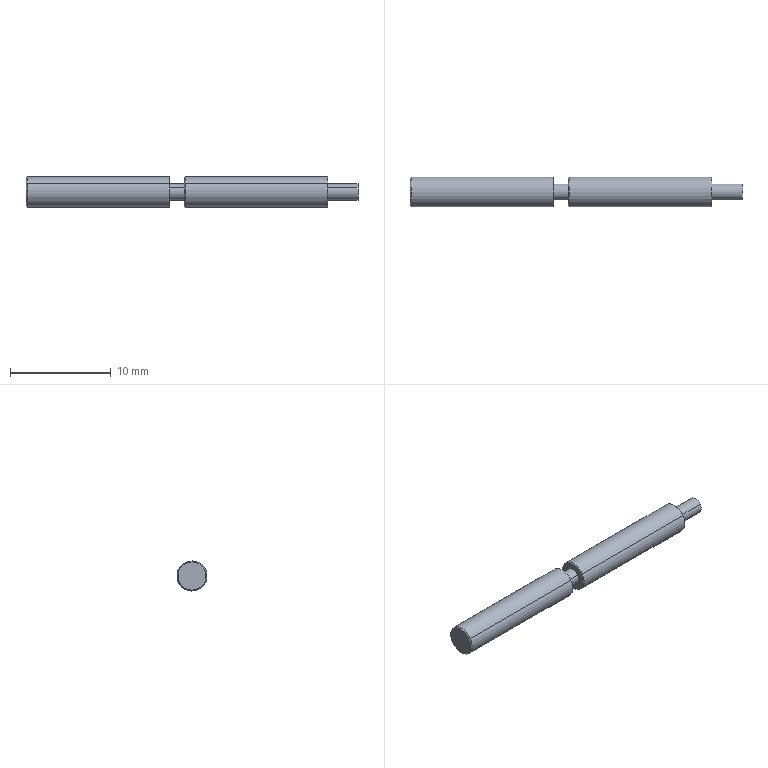Component | SolidWorks | SliderScrew2-1 | 1 solid | 17 faces | box 33 x 3 x 3 mm | volume 210 mm3 | cylinder 8 | plane 5 | cone 4 | commonest cylinder face diameters 1.6 x4 3 x4
build123d program:
from build123d import *

# Parameters (mm, degrees)
SKETCH1_R           = 1.5
BOSS_EXTRUDE1_DEPTH = 15
CHAMFER1_SIZE       = 0.1
SKETCH2_R           = 1.5
SKETCH2_R_2         = 0.8
CUT_EXTRUDE1_DEPTH  = 0.75
CHAMFER2_SIZE       = 0.1
SKETCH3_R           = 0.8
BOSS_EXTRUDE2_DEPTH = 3


with BuildPart() as part:
    # Sketch1 → Boss-Extrude1 (new, symmetric)
    with BuildSketch(Plane.XY):
        Circle(SKETCH1_R)
    extrude(amount=BOSS_EXTRUDE1_DEPTH, both=True)

    # Chamfer1
    chamfer1_edges = [part.edges().sort_by_distance(p)[0] for p in [
        (-1.5, 0, -15),
    ]]
    chamfer(chamfer1_edges, length=CHAMFER1_SIZE)

    # Sketch2 → Cut-Extrude1 (cut, symmetric)
    with BuildSketch(Plane.XY):
        Circle(SKETCH2_R)
        Circle(SKETCH2_R_2, mode=Mode.SUBTRACT)
    extrude(amount=CUT_EXTRUDE1_DEPTH, both=True, mode=Mode.SUBTRACT)

    # Chamfer2
    chamfer2_edges = [part.edges().sort_by_distance(p)[0] for p in [
        (-1.5, 0, 0.75),
    ]]
    chamfer(chamfer2_edges, length=CHAMFER2_SIZE)

    # Sketch3 → Boss-Extrude2 (add)
    with BuildSketch(Plane.XY.offset(15)):
        Circle(SKETCH3_R)
    extrude(amount=BOSS_EXTRUDE2_DEPTH)


solid = part.part

# Placed as in the assembly
solid = solid.moved(Location((-5.981, 33.561, 233.566), (0, 90, 0)))
STEP:
#1=COLOUR_RGB('',0.7922,0.8196,0.9333);
#2=FILL_AREA_STYLE_COLOUR('',#1);
#3=FILL_AREA_STYLE('',(#2));
#4=SURFACE_STYLE_FILL_AREA(#3);
#5=SURFACE_SIDE_STYLE('',(#4));
#6=SURFACE_STYLE_USAGE(.BOTH.,#5);
#7=PRESENTATION_STYLE_ASSIGNMENT((#6));
#8=CARTESIAN_POINT('',(0.4732,1.295,9.213));
#9=VERTEX_POINT('',#8);
#10=CARTESIAN_POINT('',(0.4732,1.347,9.178));
#11=VERTEX_POINT('',#10);
#12=CARTESIAN_POINT('',(0.4732,1.321,9.196));
#13=DIRECTION('',(1.,0.,-0.));
#14=DIRECTION('',(0.,-0.8262,0.5634));
#15=AXIS2_PLACEMENT_3D('',#12,#13,#14);
#16=CIRCLE('',#15,0.0315);
#17=EDGE_CURVE('',#9,#11,#16,.T.);
#18=ORIENTED_EDGE('',*,*,#17,.F.);
#19=CARTESIAN_POINT('',(0.3551,1.295,9.213));
#20=VERTEX_POINT('',#19);
#21=CARTESIAN_POINT('',(0.4732,1.295,9.213));
#22=DIRECTION('',(-1.,-0.,0.));
#23=VECTOR('',#22,39.37);
#24=LINE('',#21,#23);
#25=EDGE_CURVE('',#9,#20,#24,.T.);
#26=ORIENTED_EDGE('',*,*,#25,.T.);
#27=CARTESIAN_POINT('',(0.3551,1.347,9.178));
#28=VERTEX_POINT('',#27);
#29=CARTESIAN_POINT('',(0.3551,1.321,9.196));
#30=DIRECTION('',(1.,0.,-0.));
#31=DIRECTION('',(0.,-0.8262,0.5634));
#32=AXIS2_PLACEMENT_3D('',#29,#30,#31);
#33=CIRCLE('',#32,0.0315);
#34=EDGE_CURVE('',#20,#28,#33,.T.);
#35=ORIENTED_EDGE('',*,*,#34,.T.);
#36=CARTESIAN_POINT('',(0.4732,1.347,9.178));
#37=DIRECTION('',(-1.,-0.,0.));
#38=VECTOR('',#37,39.37);
#39=LINE('',#36,#38);
#40=EDGE_CURVE('',#11,#28,#39,.T.);
#41=ORIENTED_EDGE('',*,*,#40,.F.);
#42=EDGE_LOOP('',(#18,#26,#35,#41));
#43=FACE_OUTER_BOUND('',#42,.T.);
#44=CARTESIAN_POINT('',(0.4732,1.321,9.196));
#45=DIRECTION('',(-1.,-0.,0.));
#46=DIRECTION('',(0.,0.8262,-0.5634));
#47=AXIS2_PLACEMENT_3D('',#44,#45,#46);
#48=CYLINDRICAL_SURFACE('',#47,0.0315);
#49=ADVANCED_FACE('',(#43),#48,.T.);
#50=CARTESIAN_POINT('',(-0.2059,1.367,9.164));
#51=VERTEX_POINT('',#50);
#52=CARTESIAN_POINT('',(-0.2059,1.276,9.227));
#53=VERTEX_POINT('',#52);
#54=CARTESIAN_POINT('',(-0.2059,1.321,9.196));
#55=DIRECTION('',(-1.,-0.,0.));
#56=DIRECTION('',(0.,-0.8262,0.5634));
#57=AXIS2_PLACEMENT_3D('',#54,#55,#56);
#58=CIRCLE('',#57,0.05512);
#59=EDGE_CURVE('',#51,#53,#58,.T.);
#60=ORIENTED_EDGE('',*,*,#59,.F.);
#61=CARTESIAN_POINT('',(-0.202,1.37,9.162));
#62=VERTEX_POINT('',#61);
#63=CARTESIAN_POINT('',(-0.202,1.37,9.162));
#64=DIRECTION('',(0.7071,0.5842,-0.3984));
#65=VECTOR('',#64,39.37);
#66=LINE('',#63,#65);
#67=EDGE_CURVE('',#51,#62,#66,.T.);
#68=ORIENTED_EDGE('',*,*,#67,.T.);
#69=CARTESIAN_POINT('',(-0.202,1.272,9.229));
#70=VERTEX_POINT('',#69);
#71=CARTESIAN_POINT('',(-0.202,1.321,9.196));
#72=DIRECTION('',(1.,0.,-0.));
#73=DIRECTION('',(0.,-0.8262,0.5634));
#74=AXIS2_PLACEMENT_3D('',#71,#72,#73);
#75=CIRCLE('',#74,0.05906);
#76=EDGE_CURVE('',#70,#62,#75,.T.);
#77=ORIENTED_EDGE('',*,*,#76,.F.);
#78=CARTESIAN_POINT('',(-0.202,1.272,9.229));
#79=DIRECTION('',(0.7071,-0.5842,0.3984));
#80=VECTOR('',#79,39.37);
#81=LINE('',#78,#80);
#82=EDGE_CURVE('',#53,#70,#81,.T.);
#83=ORIENTED_EDGE('',*,*,#82,.F.);
#84=EDGE_LOOP('',(#60,#68,#77,#83));
#85=FACE_OUTER_BOUND('',#84,.T.);
#86=CARTESIAN_POINT('',(-0.202,1.321,9.196));
#87=DIRECTION('',(1.,0.,-0.));
#88=DIRECTION('',(0.,-0.8262,0.5634));
#89=AXIS2_PLACEMENT_3D('',#86,#87,#88);
#90=CONICAL_SURFACE('',#89,0.05906,0.7854);
#91=ADVANCED_FACE('',(#85),#90,.T.);
#92=CARTESIAN_POINT('',(0.3551,1.272,9.229));
#93=VERTEX_POINT('',#92);
#94=CARTESIAN_POINT('',(0.3551,1.37,9.162));
#95=VERTEX_POINT('',#94);
#96=CARTESIAN_POINT('',(0.3551,1.321,9.196));
#97=DIRECTION('',(1.,0.,-0.));
#98=DIRECTION('',(0.,-0.8262,0.5634));
#99=AXIS2_PLACEMENT_3D('',#96,#97,#98);
#100=CIRCLE('',#99,0.05906);
#101=EDGE_CURVE('',#93,#95,#100,.T.);
#102=ORIENTED_EDGE('',*,*,#101,.F.);
#103=CARTESIAN_POINT('',(0.3551,1.272,9.229));
#104=DIRECTION('',(-1.,-0.,0.));
#105=VECTOR('',#104,39.37);
#106=LINE('',#103,#105);
#107=EDGE_CURVE('',#93,#70,#106,.T.);
#108=ORIENTED_EDGE('',*,*,#107,.T.);
#109=ORIENTED_EDGE('',*,*,#76,.T.);
#110=CARTESIAN_POINT('',(0.3551,1.37,9.162));
#111=DIRECTION('',(-1.,-0.,0.));
#112=VECTOR('',#111,39.37);
#113=LINE('',#110,#112);
#114=EDGE_CURVE('',#95,#62,#113,.T.);
#115=ORIENTED_EDGE('',*,*,#114,.F.);
#116=EDGE_LOOP('',(#102,#108,#109,#115));
#117=FACE_OUTER_BOUND('',#116,.T.);
#118=CARTESIAN_POINT('',(0.3551,1.321,9.196));
#119=DIRECTION('',(-1.,-0.,0.));
#120=DIRECTION('',(-0.,0.8262,-0.5634));
#121=AXIS2_PLACEMENT_3D('',#118,#119,#120);
#122=CYLINDRICAL_SURFACE('',#121,0.05906);
#123=ADVANCED_FACE('',(#117),#122,.T.);
#124=CARTESIAN_POINT('',(-0.265,1.295,9.213));
#125=VERTEX_POINT('',#124);
#126=CARTESIAN_POINT('',(-0.265,1.347,9.178));
#127=VERTEX_POINT('',#126);
#128=CARTESIAN_POINT('',(-0.265,1.321,9.196));
#129=DIRECTION('',(1.,0.,-0.));
#130=DIRECTION('',(0.,-0.8262,0.5634));
#131=AXIS2_PLACEMENT_3D('',#128,#129,#130);
#132=CIRCLE('',#131,0.0315);
#133=EDGE_CURVE('',#125,#127,#132,.T.);
#134=ORIENTED_EDGE('',*,*,#133,.T.);
#135=CARTESIAN_POINT('',(-0.2059,1.347,9.178));
#136=VERTEX_POINT('',#135);
#137=CARTESIAN_POINT('',(-0.265,1.347,9.178));
#138=DIRECTION('',(1.,0.,-0.));
#139=VECTOR('',#138,39.37);
#140=LINE('',#137,#139);
#141=EDGE_CURVE('',#127,#136,#140,.T.);
#142=ORIENTED_EDGE('',*,*,#141,.T.);
#143=CARTESIAN_POINT('',(-0.2059,1.295,9.213));
#144=VERTEX_POINT('',#143);
#145=CARTESIAN_POINT('',(-0.2059,1.321,9.196));
#146=DIRECTION('',(1.,0.,-0.));
#147=DIRECTION('',(0.,-0.8262,0.5634));
#148=AXIS2_PLACEMENT_3D('',#145,#146,#147);
#149=CIRCLE('',#148,0.0315);
#150=EDGE_CURVE('',#144,#136,#149,.T.);
#151=ORIENTED_EDGE('',*,*,#150,.F.);
#152=CARTESIAN_POINT('',(-0.265,1.295,9.213));
#153=DIRECTION('',(1.,0.,-0.));
#154=VECTOR('',#153,39.37);
#155=LINE('',#152,#154);
#156=EDGE_CURVE('',#125,#144,#155,.T.);
#157=ORIENTED_EDGE('',*,*,#156,.F.);
#158=EDGE_LOOP('',(#134,#142,#151,#157));
#159=FACE_OUTER_BOUND('',#158,.T.);
#160=CARTESIAN_POINT('',(-0.265,1.321,9.196));
#161=DIRECTION('',(1.,0.,-0.));
#162=DIRECTION('',(0.,-0.8262,0.5634));
#163=AXIS2_PLACEMENT_3D('',#160,#161,#162);
#164=CYLINDRICAL_SURFACE('',#163,0.0315);
#165=ADVANCED_FACE('',(#159),#164,.T.);
#166=CARTESIAN_POINT('',(-0.826,1.367,9.164));
#167=VERTEX_POINT('',#166);
#168=CARTESIAN_POINT('',(-0.826,1.276,9.227));
#169=VERTEX_POINT('',#168);
#170=CARTESIAN_POINT('',(-0.826,1.321,9.196));
#171=DIRECTION('',(-1.,-0.,0.));
#172=DIRECTION('',(0.,-0.8262,0.5634));
#173=AXIS2_PLACEMENT_3D('',#170,#171,#172);
#174=CIRCLE('',#173,0.05512);
#175=EDGE_CURVE('',#167,#169,#174,.T.);
#176=ORIENTED_EDGE('',*,*,#175,.F.);
#177=CARTESIAN_POINT('',(-0.8221,1.37,9.162));
#178=VERTEX_POINT('',#177);
#179=CARTESIAN_POINT('',(-0.8221,1.37,9.162));
#180=DIRECTION('',(0.7071,0.5842,-0.3984));
#181=VECTOR('',#180,39.37);
#182=LINE('',#179,#181);
#183=EDGE_CURVE('',#167,#178,#182,.T.);
#184=ORIENTED_EDGE('',*,*,#183,.T.);
#185=CARTESIAN_POINT('',(-0.8221,1.272,9.229));
#186=VERTEX_POINT('',#185);
#187=CARTESIAN_POINT('',(-0.8221,1.321,9.196));
#188=DIRECTION('',(1.,0.,-0.));
#189=DIRECTION('',(0.,-0.8262,0.5634));
#190=AXIS2_PLACEMENT_3D('',#187,#188,#189);
#191=CIRCLE('',#190,0.05906);
#192=EDGE_CURVE('',#186,#178,#191,.T.);
#193=ORIENTED_EDGE('',*,*,#192,.F.);
#194=CARTESIAN_POINT('',(-0.8221,1.272,9.229));
#195=DIRECTION('',(0.7071,-0.5842,0.3984));
#196=VECTOR('',#195,39.37);
#197=LINE('',#194,#196);
#198=EDGE_CURVE('',#169,#186,#197,.T.);
#199=ORIENTED_EDGE('',*,*,#198,.F.);
#200=EDGE_LOOP('',(#176,#184,#193,#199));
#201=FACE_OUTER_BOUND('',#200,.T.);
#202=CARTESIAN_POINT('',(-0.8221,1.321,9.196));
#203=DIRECTION('',(1.,0.,-0.));
#204=DIRECTION('',(0.,-0.8262,0.5634));
#205=AXIS2_PLACEMENT_3D('',#202,#203,#204);
#206=CONICAL_SURFACE('',#205,0.05906,0.7854);
#207=ADVANCED_FACE('',(#201),#206,.T.);
#208=CARTESIAN_POINT('',(-0.265,1.272,9.229));
#209=VERTEX_POINT('',#208);
#210=CARTESIAN_POINT('',(-0.265,1.37,9.162));
#211=VERTEX_POINT('',#210);
#212=CARTESIAN_POINT('',(-0.265,1.321,9.196));
#213=DIRECTION('',(1.,0.,-0.));
#214=DIRECTION('',(0.,-0.8262,0.5634));
#215=AXIS2_PLACEMENT_3D('',#212,#213,#214);
#216=CIRCLE('',#215,0.05906);
#217=EDGE_CURVE('',#209,#211,#216,.T.);
#218=ORIENTED_EDGE('',*,*,#217,.F.);
#219=CARTESIAN_POINT('',(0.3551,1.272,9.229));
#220=DIRECTION('',(-1.,-0.,0.));
#221=VECTOR('',#220,39.37);
#222=LINE('',#219,#221);
#223=EDGE_CURVE('',#209,#186,#222,.T.);
#224=ORIENTED_EDGE('',*,*,#223,.T.);
#225=ORIENTED_EDGE('',*,*,#192,.T.);
#226=CARTESIAN_POINT('',(0.3551,1.37,9.162));
#227=DIRECTION('',(-1.,-0.,0.));
#228=VECTOR('',#227,39.37);
#229=LINE('',#226,#228);
#230=EDGE_CURVE('',#211,#178,#229,.T.);
#231=ORIENTED_EDGE('',*,*,#230,.F.);
#232=EDGE_LOOP('',(#218,#224,#225,#231));
#233=FACE_OUTER_BOUND('',#232,.T.);
#234=CARTESIAN_POINT('',(0.3551,1.321,9.196));
#235=DIRECTION('',(-1.,-0.,0.));
#236=DIRECTION('',(-0.,0.8262,-0.5634));
#237=AXIS2_PLACEMENT_3D('',#234,#235,#236);
#238=CYLINDRICAL_SURFACE('',#237,0.05906);
#239=ADVANCED_FACE('',(#233),#238,.T.);
#240=ORIENTED_EDGE('',*,*,#223,.F.);
#241=CARTESIAN_POINT('',(-0.265,1.321,9.196));
#242=DIRECTION('',(1.,0.,-0.));
#243=DIRECTION('',(0.,-0.8262,0.5634));
#244=AXIS2_PLACEMENT_3D('',#241,#242,#243);
#245=CIRCLE('',#244,0.05906);
#246=EDGE_CURVE('',#211,#209,#245,.T.);
#247=ORIENTED_EDGE('',*,*,#246,.F.);
#248=ORIENTED_EDGE('',*,*,#230,.T.);
#249=CARTESIAN_POINT('',(-0.8221,1.321,9.196));
#250=DIRECTION('',(1.,0.,-0.));
#251=DIRECTION('',(0.,-0.8262,0.5634));
#252=AXIS2_PLACEMENT_3D('',#249,#250,#251);
#253=CIRCLE('',#252,0.05906);
#254=EDGE_CURVE('',#178,#186,#253,.T.);
#255=ORIENTED_EDGE('',*,*,#254,.T.);
#256=EDGE_LOOP('',(#240,#247,#248,#255));
#257=FACE_OUTER_BOUND('',#256,.T.);
#258=CARTESIAN_POINT('',(0.3551,1.321,9.196));
#259=DIRECTION('',(-1.,-0.,0.));
#260=DIRECTION('',(-0.,0.8262,-0.5634));
#261=AXIS2_PLACEMENT_3D('',#258,#259,#260);
#262=CYLINDRICAL_SURFACE('',#261,0.05906);
#263=ADVANCED_FACE('',(#257),#262,.T.);
#264=CARTESIAN_POINT('',(-0.826,1.321,9.196));
#265=DIRECTION('',(-1.,-0.,0.));
#266=DIRECTION('',(0.,-0.8262,0.5634));
#267=AXIS2_PLACEMENT_3D('',#264,#265,#266);
#268=CIRCLE('',#267,0.05512);
#269=EDGE_CURVE('',#169,#167,#268,.T.);
#270=ORIENTED_EDGE('',*,*,#269,.T.);
#271=ORIENTED_EDGE('',*,*,#175,.T.);
#272=EDGE_LOOP('',(#270,#271));
#273=FACE_OUTER_BOUND('',#272,.T.);
#274=CARTESIAN_POINT('',(-0.826,1.321,9.196));
#275=DIRECTION('',(1.,0.,-0.));
#276=DIRECTION('',(0.,-0.8262,0.5634));
#277=AXIS2_PLACEMENT_3D('',#274,#275,#276);
#278=PLANE('',#277);
#279=ADVANCED_FACE('',(#273),#278,.F.);
#280=ORIENTED_EDGE('',*,*,#183,.F.);
#281=ORIENTED_EDGE('',*,*,#269,.F.);
#282=ORIENTED_EDGE('',*,*,#198,.T.);
#283=ORIENTED_EDGE('',*,*,#254,.F.);
#284=EDGE_LOOP('',(#280,#281,#282,#283));
#285=FACE_OUTER_BOUND('',#284,.T.);
#286=CARTESIAN_POINT('',(-0.8221,1.321,9.196));
#287=DIRECTION('',(1.,0.,-0.));
#288=DIRECTION('',(0.,-0.8262,0.5634));
#289=AXIS2_PLACEMENT_3D('',#286,#287,#288);
#290=CONICAL_SURFACE('',#289,0.05906,0.7854);
#291=ADVANCED_FACE('',(#285),#290,.T.);
#292=ORIENTED_EDGE('',*,*,#133,.F.);
#293=CARTESIAN_POINT('',(-0.265,1.321,9.196));
#294=DIRECTION('',(1.,0.,-0.));
#295=DIRECTION('',(0.,-0.8262,0.5634));
#296=AXIS2_PLACEMENT_3D('',#293,#294,#295);
#297=CIRCLE('',#296,0.0315);
#298=EDGE_CURVE('',#127,#125,#297,.T.);
#299=ORIENTED_EDGE('',*,*,#298,.F.);
#300=EDGE_LOOP('',(#292,#299));
#301=FACE_BOUND('',#300,.T.);
#302=ORIENTED_EDGE('',*,*,#246,.T.);
#303=ORIENTED_EDGE('',*,*,#217,.T.);
#304=EDGE_LOOP('',(#302,#303));
#305=FACE_OUTER_BOUND('',#304,.T.);
#306=CARTESIAN_POINT('',(-0.265,1.321,9.196));
#307=DIRECTION('',(1.,0.,-0.));
#308=DIRECTION('',(0.,-0.8262,0.5634));
#309=AXIS2_PLACEMENT_3D('',#306,#307,#308);
#310=PLANE('',#309);
#311=ADVANCED_FACE('',(#301,#305),#310,.T.);
#312=CARTESIAN_POINT('',(-0.2059,1.321,9.196));
#313=DIRECTION('',(-1.,-0.,0.));
#314=DIRECTION('',(0.,-0.8262,0.5634));
#315=AXIS2_PLACEMENT_3D('',#312,#313,#314);
#316=CIRCLE('',#315,0.05512);
#317=EDGE_CURVE('',#53,#51,#316,.T.);
#318=ORIENTED_EDGE('',*,*,#317,.T.);
#319=ORIENTED_EDGE('',*,*,#59,.T.);
#320=EDGE_LOOP('',(#318,#319));
#321=FACE_OUTER_BOUND('',#320,.T.);
#322=ORIENTED_EDGE('',*,*,#150,.T.);
#323=CARTESIAN_POINT('',(-0.2059,1.321,9.196));
#324=DIRECTION('',(1.,0.,-0.));
#325=DIRECTION('',(0.,-0.8262,0.5634));
#326=AXIS2_PLACEMENT_3D('',#323,#324,#325);
#327=CIRCLE('',#326,0.0315);
#328=EDGE_CURVE('',#136,#144,#327,.T.);
#329=ORIENTED_EDGE('',*,*,#328,.T.);
#330=EDGE_LOOP('',(#322,#329));
#331=FACE_BOUND('',#330,.T.);
#332=CARTESIAN_POINT('',(-0.2059,1.321,9.196));
#333=DIRECTION('',(1.,0.,-0.));
#334=DIRECTION('',(0.,-0.8262,0.5634));
#335=AXIS2_PLACEMENT_3D('',#332,#333,#334);
#336=PLANE('',#335);
#337=ADVANCED_FACE('',(#321,#331),#336,.F.);
#338=ORIENTED_EDGE('',*,*,#141,.F.);
#339=ORIENTED_EDGE('',*,*,#298,.T.);
#340=ORIENTED_EDGE('',*,*,#156,.T.);
#341=ORIENTED_EDGE('',*,*,#328,.F.);
#342=EDGE_LOOP('',(#338,#339,#340,#341));
#343=FACE_OUTER_BOUND('',#342,.T.);
#344=CARTESIAN_POINT('',(-0.265,1.321,9.196));
#345=DIRECTION('',(1.,0.,-0.));
#346=DIRECTION('',(0.,-0.8262,0.5634));
#347=AXIS2_PLACEMENT_3D('',#344,#345,#346);
#348=CYLINDRICAL_SURFACE('',#347,0.0315);
#349=ADVANCED_FACE('',(#343),#348,.T.);
#350=CARTESIAN_POINT('',(0.3551,1.321,9.196));
#351=DIRECTION('',(1.,0.,-0.));
#352=DIRECTION('',(0.,-0.8262,0.5634));
#353=AXIS2_PLACEMENT_3D('',#350,#351,#352);
#354=CIRCLE('',#353,0.0315);
#355=EDGE_CURVE('',#28,#20,#354,.T.);
#356=ORIENTED_EDGE('',*,*,#355,.F.);
#357=ORIENTED_EDGE('',*,*,#34,.F.);
#358=EDGE_LOOP('',(#356,#357));
#359=FACE_BOUND('',#358,.T.);
#360=CARTESIAN_POINT('',(0.3551,1.321,9.196));
#361=DIRECTION('',(1.,0.,-0.));
#362=DIRECTION('',(0.,-0.8262,0.5634));
#363=AXIS2_PLACEMENT_3D('',#360,#361,#362);
#364=CIRCLE('',#363,0.05906);
#365=EDGE_CURVE('',#95,#93,#364,.T.);
#366=ORIENTED_EDGE('',*,*,#365,.T.);
#367=ORIENTED_EDGE('',*,*,#101,.T.);
#368=EDGE_LOOP('',(#366,#367));
#369=FACE_OUTER_BOUND('',#368,.T.);
#370=CARTESIAN_POINT('',(0.3551,1.321,9.196));
#371=DIRECTION('',(1.,0.,-0.));
#372=DIRECTION('',(0.,-0.8262,0.5634));
#373=AXIS2_PLACEMENT_3D('',#370,#371,#372);
#374=PLANE('',#373);
#375=ADVANCED_FACE('',(#359,#369),#374,.T.);
#376=ORIENTED_EDGE('',*,*,#107,.F.);
#377=ORIENTED_EDGE('',*,*,#365,.F.);
#378=ORIENTED_EDGE('',*,*,#114,.T.);
#379=CARTESIAN_POINT('',(-0.202,1.321,9.196));
#380=DIRECTION('',(1.,0.,-0.));
#381=DIRECTION('',(0.,-0.8262,0.5634));
#382=AXIS2_PLACEMENT_3D('',#379,#380,#381);
#383=CIRCLE('',#382,0.05906);
#384=EDGE_CURVE('',#62,#70,#383,.T.);
#385=ORIENTED_EDGE('',*,*,#384,.T.);
#386=EDGE_LOOP('',(#376,#377,#378,#385));
#387=FACE_OUTER_BOUND('',#386,.T.);
#388=CARTESIAN_POINT('',(0.3551,1.321,9.196));
#389=DIRECTION('',(-1.,-0.,0.));
#390=DIRECTION('',(-0.,0.8262,-0.5634));
#391=AXIS2_PLACEMENT_3D('',#388,#389,#390);
#392=CYLINDRICAL_SURFACE('',#391,0.05906);
#393=ADVANCED_FACE('',(#387),#392,.T.);
#394=ORIENTED_EDGE('',*,*,#67,.F.);
#395=ORIENTED_EDGE('',*,*,#317,.F.);
#396=ORIENTED_EDGE('',*,*,#82,.T.);
#397=ORIENTED_EDGE('',*,*,#384,.F.);
#398=EDGE_LOOP('',(#394,#395,#396,#397));
#399=FACE_OUTER_BOUND('',#398,.T.);
#400=CARTESIAN_POINT('',(-0.202,1.321,9.196));
#401=DIRECTION('',(1.,0.,-0.));
#402=DIRECTION('',(0.,-0.8262,0.5634));
#403=AXIS2_PLACEMENT_3D('',#400,#401,#402);
#404=CONICAL_SURFACE('',#403,0.05906,0.7854);
#405=ADVANCED_FACE('',(#399),#404,.T.);
#406=ORIENTED_EDGE('',*,*,#25,.F.);
#407=CARTESIAN_POINT('',(0.4732,1.321,9.196));
#408=DIRECTION('',(1.,0.,-0.));
#409=DIRECTION('',(0.,-0.8262,0.5634));
#410=AXIS2_PLACEMENT_3D('',#407,#408,#409);
#411=CIRCLE('',#410,0.0315);
#412=EDGE_CURVE('',#11,#9,#411,.T.);
#413=ORIENTED_EDGE('',*,*,#412,.F.);
#414=ORIENTED_EDGE('',*,*,#40,.T.);
#415=ORIENTED_EDGE('',*,*,#355,.T.);
#416=EDGE_LOOP('',(#406,#413,#414,#415));
#417=FACE_OUTER_BOUND('',#416,.T.);
#418=CARTESIAN_POINT('',(0.4732,1.321,9.196));
#419=DIRECTION('',(-1.,-0.,0.));
#420=DIRECTION('',(0.,0.8262,-0.5634));
#421=AXIS2_PLACEMENT_3D('',#418,#419,#420);
#422=CYLINDRICAL_SURFACE('',#421,0.0315);
#423=ADVANCED_FACE('',(#417),#422,.T.);
#424=ORIENTED_EDGE('',*,*,#412,.T.);
#425=ORIENTED_EDGE('',*,*,#17,.T.);
#426=EDGE_LOOP('',(#424,#425));
#427=FACE_OUTER_BOUND('',#426,.T.);
#428=CARTESIAN_POINT('',(0.4732,1.321,9.196));
#429=DIRECTION('',(1.,0.,-0.));
#430=DIRECTION('',(0.,-0.8262,0.5634));
#431=AXIS2_PLACEMENT_3D('',#428,#429,#430);
#432=PLANE('',#431);
#433=ADVANCED_FACE('',(#427),#432,.T.);
#434=CLOSED_SHELL('',(#49,#91,#123,#165,#207,#239,#263,#279,#291,#311,#337,#349,#375,#393,#405,#423,#433));
#435=MANIFOLD_SOLID_BREP('',#434);
#436=STYLED_ITEM('',(#7),#435);
#437=PRESENTATION_LAYER_ASSIGNMENT('','',(#436));
#438=CARTESIAN_POINT('',(0.,0.,0.));
#439=DIRECTION('',(0.,0.,1.));
#440=DIRECTION('',(1.,0.,0.));
#441=AXIS2_PLACEMENT_3D('',#438,#439,#440);
#442=(LENGTH_UNIT()NAMED_UNIT(*)SI_UNIT($,.METRE.));
#443=LENGTH_MEASURE_WITH_UNIT(LENGTH_MEASURE(0.0254),#442);
#444=DIMENSIONAL_EXPONENTS(1.,0.,0.,0.,0.,0.,0.);
#445=(CONVERSION_BASED_UNIT('',#443)LENGTH_UNIT()NAMED_UNIT(#444));
#446=UNCERTAINTY_MEASURE_WITH_UNIT(LENGTH_MEASURE(0.00001),#445,'','');
#447=(NAMED_UNIT(*)PLANE_ANGLE_UNIT()SI_UNIT($,.RADIAN.));
#448=(NAMED_UNIT(*)SI_UNIT($,.STERADIAN.)SOLID_ANGLE_UNIT());
#449=(GEOMETRIC_REPRESENTATION_CONTEXT(3)GLOBAL_UNCERTAINTY_ASSIGNED_CONTEXT((#446))GLOBAL_UNIT_ASSIGNED_CONTEXT((#445,#447,#448))REPRESENTATION_CONTEXT('',''));
#450=ADVANCED_BREP_SHAPE_REPRESENTATION('',(#435,#441),#449);
#451=(LENGTH_UNIT()NAMED_UNIT(*)SI_UNIT($,.METRE.));
#452=LENGTH_MEASURE_WITH_UNIT(LENGTH_MEASURE(0.0254),#451);
#453=DIMENSIONAL_EXPONENTS(1.,0.,0.,0.,0.,0.,0.);
#454=(CONVERSION_BASED_UNIT('',#452)LENGTH_UNIT()NAMED_UNIT(#453));
#455=UNCERTAINTY_MEASURE_WITH_UNIT(LENGTH_MEASURE(0.00001),#454,'','');
#456=(NAMED_UNIT(*)PLANE_ANGLE_UNIT()SI_UNIT($,.RADIAN.));
#457=(NAMED_UNIT(*)SI_UNIT($,.STERADIAN.)SOLID_ANGLE_UNIT());
#458=(GEOMETRIC_REPRESENTATION_CONTEXT(3)GLOBAL_UNCERTAINTY_ASSIGNED_CONTEXT((#455))GLOBAL_UNIT_ASSIGNED_CONTEXT((#454,#456,#457))REPRESENTATION_CONTEXT('',''));
#459=MECHANICAL_DESIGN_GEOMETRIC_PRESENTATION_REPRESENTATION('',(#436),#458);